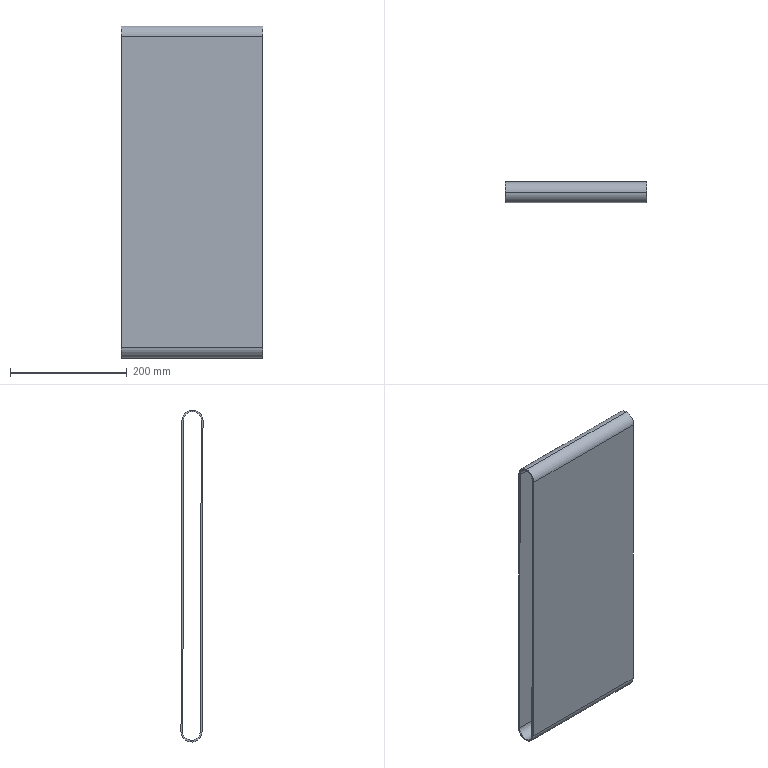Component | SolidWorks | Part7-1 | 1 solid | 12 faces | box 242 x 37.75 x 568.56 mm | volume 848551 mm3 | cylinder 6 | plane 6 | commonest cylinder face diameters 30 x3 36 x3
build123d program:
from build123d import *

# Parameters (mm, degrees)
EXTRUDE_THIN1_DEPTH = 121


with BuildPart() as part:
    # Sketch1 → Extrude-Thin1 (new, symmetric)
    with BuildSketch(Plane.XY):
        with BuildLine():
            Line((2289.339, 197.876), (1756.777, 196.124))
            ThreePointArc((1756.777, 196.124), (1738.718, 214.065), (1756.658, 232.124))
            Line((1756.658, 232.124), (2289.22, 233.876))
            ThreePointArc((2289.22, 233.876), (2307.279, 215.935), (2289.339, 197.876))
        make_face()
        with BuildLine():
            Line((2289.329, 200.876), (1756.767, 199.124))
            ThreePointArc((1756.767, 199.124), (1741.718, 214.075), (1756.668, 229.124))
            Line((1756.668, 229.124), (2289.23, 230.876))
            ThreePointArc((2289.23, 230.876), (2304.279, 215.925), (2289.329, 200.876))
        make_face(mode=Mode.SUBTRACT)
    extrude(amount=EXTRUDE_THIN1_DEPTH, both=True)


solid = part.part

# Placed as in the assembly
solid = solid.moved(Location((0, 0, -143.093), (0, 90, 0)))
STEP:
#1=CARTESIAN_POINT('',(4.764,9.021,-74.794));
#2=VERTEX_POINT('',#1);
#3=CARTESIAN_POINT('',(4.764,8.43,-74.205));
#4=VERTEX_POINT('',#3);
#5=CARTESIAN_POINT('',(4.764,8.43,-74.796));
#6=DIRECTION('',(1.,0.,0.));
#7=DIRECTION('',(0.,0.,-1.));
#8=AXIS2_PLACEMENT_3D('',#5,#6,#7);
#9=CIRCLE('',#8,0.5906);
#10=EDGE_CURVE('',#2,#4,#9,.T.);
#11=ORIENTED_EDGE('',*,*,#10,.T.);
#12=CARTESIAN_POINT('',(-4.764,8.43,-74.205));
#13=VERTEX_POINT('',#12);
#14=CARTESIAN_POINT('',(4.764,8.43,-74.205));
#15=DIRECTION('',(-1.,0.,0.));
#16=VECTOR('',#15,39.37);
#17=LINE('',#14,#16);
#18=EDGE_CURVE('',#4,#13,#17,.T.);
#19=ORIENTED_EDGE('',*,*,#18,.T.);
#20=CARTESIAN_POINT('',(-4.764,9.021,-74.794));
#21=VERTEX_POINT('',#20);
#22=CARTESIAN_POINT('',(-4.764,8.43,-74.796));
#23=DIRECTION('',(1.,0.,0.));
#24=DIRECTION('',(0.,0.,-1.));
#25=AXIS2_PLACEMENT_3D('',#22,#23,#24);
#26=CIRCLE('',#25,0.5906);
#27=EDGE_CURVE('',#21,#13,#26,.T.);
#28=ORIENTED_EDGE('',*,*,#27,.F.);
#29=CARTESIAN_POINT('',(4.764,9.021,-74.794));
#30=DIRECTION('',(-1.,0.,0.));
#31=VECTOR('',#30,39.37);
#32=LINE('',#29,#31);
#33=EDGE_CURVE('',#2,#21,#32,.T.);
#34=ORIENTED_EDGE('',*,*,#33,.F.);
#35=EDGE_LOOP('',(#11,#19,#28,#34));
#36=FACE_OUTER_BOUND('',#35,.T.);
#37=CARTESIAN_POINT('',(4.764,8.43,-74.796));
#38=DIRECTION('',(-1.,0.,0.));
#39=DIRECTION('',(0.,0.,1.));
#40=AXIS2_PLACEMENT_3D('',#37,#38,#39);
#41=CYLINDRICAL_SURFACE('',#40,0.5906);
#42=ADVANCED_FACE('',(#36),#41,.F.);
#43=CARTESIAN_POINT('',(4.764,8.43,-74.087));
#44=VERTEX_POINT('',#43);
#45=CARTESIAN_POINT('',(4.764,7.721,-74.798));
#46=VERTEX_POINT('',#45);
#47=CARTESIAN_POINT('',(4.764,8.43,-74.796));
#48=DIRECTION('',(1.,0.,0.));
#49=DIRECTION('',(0.,0.,-1.));
#50=AXIS2_PLACEMENT_3D('',#47,#48,#49);
#51=CIRCLE('',#50,0.7087);
#52=EDGE_CURVE('',#44,#46,#51,.T.);
#53=ORIENTED_EDGE('',*,*,#52,.F.);
#54=CARTESIAN_POINT('',(-4.764,8.43,-74.087));
#55=VERTEX_POINT('',#54);
#56=CARTESIAN_POINT('',(4.764,8.43,-74.087));
#57=DIRECTION('',(-1.,0.,0.));
#58=VECTOR('',#57,39.37);
#59=LINE('',#56,#58);
#60=EDGE_CURVE('',#44,#55,#59,.T.);
#61=ORIENTED_EDGE('',*,*,#60,.T.);
#62=CARTESIAN_POINT('',(-4.764,7.721,-74.798));
#63=VERTEX_POINT('',#62);
#64=CARTESIAN_POINT('',(-4.764,8.43,-74.796));
#65=DIRECTION('',(1.,0.,0.));
#66=DIRECTION('',(0.,0.,-1.));
#67=AXIS2_PLACEMENT_3D('',#64,#65,#66);
#68=CIRCLE('',#67,0.7087);
#69=EDGE_CURVE('',#55,#63,#68,.T.);
#70=ORIENTED_EDGE('',*,*,#69,.T.);
#71=CARTESIAN_POINT('',(4.764,7.721,-74.798));
#72=DIRECTION('',(-1.,0.,0.));
#73=VECTOR('',#72,39.37);
#74=LINE('',#71,#73);
#75=EDGE_CURVE('',#46,#63,#74,.T.);
#76=ORIENTED_EDGE('',*,*,#75,.F.);
#77=EDGE_LOOP('',(#53,#61,#70,#76));
#78=FACE_OUTER_BOUND('',#77,.T.);
#79=CARTESIAN_POINT('',(4.764,8.43,-74.796));
#80=DIRECTION('',(-1.,0.,0.));
#81=DIRECTION('',(0.,0.,1.));
#82=AXIS2_PLACEMENT_3D('',#79,#80,#81);
#83=CYLINDRICAL_SURFACE('',#82,0.7087);
#84=ADVANCED_FACE('',(#78),#83,.T.);
#85=CARTESIAN_POINT('',(-4.764,7.79,-95.765));
#86=VERTEX_POINT('',#85);
#87=CARTESIAN_POINT('',(-4.764,7.494,-5.609));
#88=DIRECTION('',(0.,-0.003289,1.));
#89=VECTOR('',#88,39.37);
#90=LINE('',#87,#89);
#91=EDGE_CURVE('',#86,#63,#90,.T.);
#92=ORIENTED_EDGE('',*,*,#91,.F.);
#93=CARTESIAN_POINT('',(4.764,7.79,-95.765));
#94=VERTEX_POINT('',#93);
#95=CARTESIAN_POINT('',(4.764,7.79,-95.765));
#96=DIRECTION('',(-1.,0.,0.));
#97=VECTOR('',#96,39.37);
#98=LINE('',#95,#97);
#99=EDGE_CURVE('',#94,#86,#98,.T.);
#100=ORIENTED_EDGE('',*,*,#99,.F.);
#101=CARTESIAN_POINT('',(4.764,7.494,-5.609));
#102=DIRECTION('',(0.,-0.003289,1.));
#103=VECTOR('',#102,39.37);
#104=LINE('',#101,#103);
#105=EDGE_CURVE('',#94,#46,#104,.T.);
#106=ORIENTED_EDGE('',*,*,#105,.T.);
#107=ORIENTED_EDGE('',*,*,#75,.T.);
#108=EDGE_LOOP('',(#92,#100,#106,#107));
#109=FACE_OUTER_BOUND('',#108,.T.);
#110=CARTESIAN_POINT('',(4.764,7.494,-5.609));
#111=DIRECTION('',(0.,-1.,-0.003289));
#112=DIRECTION('',(0.,0.003289,-1.));
#113=AXIS2_PLACEMENT_3D('',#110,#111,#112);
#114=PLANE('',#113);
#115=ADVANCED_FACE('',(#109),#114,.T.);
#116=CARTESIAN_POINT('',(-4.764,9.208,-95.76));
#117=VERTEX_POINT('',#116);
#118=CARTESIAN_POINT('',(-4.764,8.499,-95.763));
#119=DIRECTION('',(1.,0.,0.));
#120=DIRECTION('',(0.,0.,-1.));
#121=AXIS2_PLACEMENT_3D('',#118,#119,#120);
#122=CIRCLE('',#121,0.7087);
#123=EDGE_CURVE('',#86,#117,#122,.T.);
#124=ORIENTED_EDGE('',*,*,#123,.T.);
#125=CARTESIAN_POINT('',(4.764,9.208,-95.76));
#126=VERTEX_POINT('',#125);
#127=CARTESIAN_POINT('',(4.764,9.208,-95.76));
#128=DIRECTION('',(-1.,0.,0.));
#129=VECTOR('',#128,39.37);
#130=LINE('',#127,#129);
#131=EDGE_CURVE('',#126,#117,#130,.T.);
#132=ORIENTED_EDGE('',*,*,#131,.F.);
#133=CARTESIAN_POINT('',(4.764,8.499,-95.763));
#134=DIRECTION('',(1.,0.,0.));
#135=DIRECTION('',(0.,0.,-1.));
#136=AXIS2_PLACEMENT_3D('',#133,#134,#135);
#137=CIRCLE('',#136,0.7087);
#138=EDGE_CURVE('',#94,#126,#137,.T.);
#139=ORIENTED_EDGE('',*,*,#138,.F.);
#140=ORIENTED_EDGE('',*,*,#99,.T.);
#141=EDGE_LOOP('',(#124,#132,#139,#140));
#142=FACE_OUTER_BOUND('',#141,.T.);
#143=CARTESIAN_POINT('',(4.764,8.499,-95.763));
#144=DIRECTION('',(-1.,0.,0.));
#145=DIRECTION('',(0.,0.,1.));
#146=AXIS2_PLACEMENT_3D('',#143,#144,#145);
#147=CYLINDRICAL_SURFACE('',#146,0.7087);
#148=ADVANCED_FACE('',(#142),#147,.T.);
#149=CARTESIAN_POINT('',(-4.764,9.139,-74.793));
#150=VERTEX_POINT('',#149);
#151=CARTESIAN_POINT('',(-4.764,8.911,-5.604));
#152=DIRECTION('',(0.,0.003289,-1.));
#153=VECTOR('',#152,39.37);
#154=LINE('',#151,#153);
#155=EDGE_CURVE('',#150,#117,#154,.T.);
#156=ORIENTED_EDGE('',*,*,#155,.F.);
#157=CARTESIAN_POINT('',(4.764,9.139,-74.793));
#158=VERTEX_POINT('',#157);
#159=CARTESIAN_POINT('',(4.764,9.139,-74.793));
#160=DIRECTION('',(-1.,0.,0.));
#161=VECTOR('',#160,39.37);
#162=LINE('',#159,#161);
#163=EDGE_CURVE('',#158,#150,#162,.T.);
#164=ORIENTED_EDGE('',*,*,#163,.F.);
#165=CARTESIAN_POINT('',(4.764,8.911,-5.604));
#166=DIRECTION('',(0.,0.003289,-1.));
#167=VECTOR('',#166,39.37);
#168=LINE('',#165,#167);
#169=EDGE_CURVE('',#158,#126,#168,.T.);
#170=ORIENTED_EDGE('',*,*,#169,.T.);
#171=ORIENTED_EDGE('',*,*,#131,.T.);
#172=EDGE_LOOP('',(#156,#164,#170,#171));
#173=FACE_OUTER_BOUND('',#172,.T.);
#174=CARTESIAN_POINT('',(4.764,8.911,-5.604));
#175=DIRECTION('',(0.,1.,0.003289));
#176=DIRECTION('',(0.,-0.003289,1.));
#177=AXIS2_PLACEMENT_3D('',#174,#175,#176);
#178=PLANE('',#177);
#179=ADVANCED_FACE('',(#173),#178,.T.);
#180=ORIENTED_EDGE('',*,*,#60,.F.);
#181=CARTESIAN_POINT('',(4.764,8.43,-74.796));
#182=DIRECTION('',(1.,0.,0.));
#183=DIRECTION('',(0.,0.,-1.));
#184=AXIS2_PLACEMENT_3D('',#181,#182,#183);
#185=CIRCLE('',#184,0.7087);
#186=EDGE_CURVE('',#158,#44,#185,.T.);
#187=ORIENTED_EDGE('',*,*,#186,.F.);
#188=ORIENTED_EDGE('',*,*,#163,.T.);
#189=CARTESIAN_POINT('',(-4.764,8.43,-74.796));
#190=DIRECTION('',(1.,0.,0.));
#191=DIRECTION('',(0.,0.,-1.));
#192=AXIS2_PLACEMENT_3D('',#189,#190,#191);
#193=CIRCLE('',#192,0.7087);
#194=EDGE_CURVE('',#150,#55,#193,.T.);
#195=ORIENTED_EDGE('',*,*,#194,.T.);
#196=EDGE_LOOP('',(#180,#187,#188,#195));
#197=FACE_OUTER_BOUND('',#196,.T.);
#198=CARTESIAN_POINT('',(4.764,8.43,-74.796));
#199=DIRECTION('',(-1.,0.,0.));
#200=DIRECTION('',(0.,0.,1.));
#201=AXIS2_PLACEMENT_3D('',#198,#199,#200);
#202=CYLINDRICAL_SURFACE('',#201,0.7087);
#203=ADVANCED_FACE('',(#197),#202,.T.);
#204=CARTESIAN_POINT('',(4.764,7.909,-95.765));
#205=VERTEX_POINT('',#204);
#206=CARTESIAN_POINT('',(4.764,7.84,-74.798));
#207=VERTEX_POINT('',#206);
#208=CARTESIAN_POINT('',(4.764,7.612,-5.609));
#209=DIRECTION('',(0.,-0.003289,1.));
#210=VECTOR('',#209,39.37);
#211=LINE('',#208,#210);
#212=EDGE_CURVE('',#205,#207,#211,.T.);
#213=ORIENTED_EDGE('',*,*,#212,.T.);
#214=CARTESIAN_POINT('',(4.764,8.43,-74.796));
#215=DIRECTION('',(1.,0.,0.));
#216=DIRECTION('',(0.,0.,-1.));
#217=AXIS2_PLACEMENT_3D('',#214,#215,#216);
#218=CIRCLE('',#217,0.5906);
#219=EDGE_CURVE('',#4,#207,#218,.T.);
#220=ORIENTED_EDGE('',*,*,#219,.F.);
#221=ORIENTED_EDGE('',*,*,#10,.F.);
#222=CARTESIAN_POINT('',(4.764,9.09,-95.761));
#223=VERTEX_POINT('',#222);
#224=CARTESIAN_POINT('',(4.764,8.793,-5.605));
#225=DIRECTION('',(0.,0.003289,-1.));
#226=VECTOR('',#225,39.37);
#227=LINE('',#224,#226);
#228=EDGE_CURVE('',#2,#223,#227,.T.);
#229=ORIENTED_EDGE('',*,*,#228,.T.);
#230=CARTESIAN_POINT('',(4.764,8.499,-95.763));
#231=DIRECTION('',(1.,0.,0.));
#232=DIRECTION('',(0.,0.,-1.));
#233=AXIS2_PLACEMENT_3D('',#230,#231,#232);
#234=CIRCLE('',#233,0.5906);
#235=EDGE_CURVE('',#205,#223,#234,.T.);
#236=ORIENTED_EDGE('',*,*,#235,.F.);
#237=EDGE_LOOP('',(#213,#220,#221,#229,#236));
#238=FACE_BOUND('',#237,.T.);
#239=ORIENTED_EDGE('',*,*,#105,.F.);
#240=ORIENTED_EDGE('',*,*,#138,.T.);
#241=ORIENTED_EDGE('',*,*,#169,.F.);
#242=ORIENTED_EDGE('',*,*,#186,.T.);
#243=ORIENTED_EDGE('',*,*,#52,.T.);
#244=EDGE_LOOP('',(#239,#240,#241,#242,#243));
#245=FACE_OUTER_BOUND('',#244,.T.);
#246=CARTESIAN_POINT('',(4.764,8.43,-74.796));
#247=DIRECTION('',(1.,0.,0.));
#248=DIRECTION('',(0.,0.,-1.));
#249=AXIS2_PLACEMENT_3D('',#246,#247,#248);
#250=PLANE('',#249);
#251=ADVANCED_FACE('',(#238,#245),#250,.T.);
#252=ORIENTED_EDGE('',*,*,#27,.T.);
#253=CARTESIAN_POINT('',(-4.764,7.84,-74.798));
#254=VERTEX_POINT('',#253);
#255=CARTESIAN_POINT('',(-4.764,8.43,-74.796));
#256=DIRECTION('',(1.,0.,0.));
#257=DIRECTION('',(0.,0.,-1.));
#258=AXIS2_PLACEMENT_3D('',#255,#256,#257);
#259=CIRCLE('',#258,0.5906);
#260=EDGE_CURVE('',#13,#254,#259,.T.);
#261=ORIENTED_EDGE('',*,*,#260,.T.);
#262=CARTESIAN_POINT('',(-4.764,7.909,-95.765));
#263=VERTEX_POINT('',#262);
#264=CARTESIAN_POINT('',(-4.764,7.612,-5.609));
#265=DIRECTION('',(0.,-0.003289,1.));
#266=VECTOR('',#265,39.37);
#267=LINE('',#264,#266);
#268=EDGE_CURVE('',#263,#254,#267,.T.);
#269=ORIENTED_EDGE('',*,*,#268,.F.);
#270=CARTESIAN_POINT('',(-4.764,9.09,-95.761));
#271=VERTEX_POINT('',#270);
#272=CARTESIAN_POINT('',(-4.764,8.499,-95.763));
#273=DIRECTION('',(1.,0.,0.));
#274=DIRECTION('',(0.,0.,-1.));
#275=AXIS2_PLACEMENT_3D('',#272,#273,#274);
#276=CIRCLE('',#275,0.5906);
#277=EDGE_CURVE('',#263,#271,#276,.T.);
#278=ORIENTED_EDGE('',*,*,#277,.T.);
#279=CARTESIAN_POINT('',(-4.764,8.793,-5.605));
#280=DIRECTION('',(0.,0.003289,-1.));
#281=VECTOR('',#280,39.37);
#282=LINE('',#279,#281);
#283=EDGE_CURVE('',#21,#271,#282,.T.);
#284=ORIENTED_EDGE('',*,*,#283,.F.);
#285=EDGE_LOOP('',(#252,#261,#269,#278,#284));
#286=FACE_BOUND('',#285,.T.);
#287=ORIENTED_EDGE('',*,*,#91,.T.);
#288=ORIENTED_EDGE('',*,*,#69,.F.);
#289=ORIENTED_EDGE('',*,*,#194,.F.);
#290=ORIENTED_EDGE('',*,*,#155,.T.);
#291=ORIENTED_EDGE('',*,*,#123,.F.);
#292=EDGE_LOOP('',(#287,#288,#289,#290,#291));
#293=FACE_OUTER_BOUND('',#292,.T.);
#294=CARTESIAN_POINT('',(-4.764,8.43,-74.796));
#295=DIRECTION('',(1.,0.,0.));
#296=DIRECTION('',(0.,0.,-1.));
#297=AXIS2_PLACEMENT_3D('',#294,#295,#296);
#298=PLANE('',#297);
#299=ADVANCED_FACE('',(#286,#293),#298,.F.);
#300=ORIENTED_EDGE('',*,*,#268,.T.);
#301=CARTESIAN_POINT('',(4.764,7.84,-74.798));
#302=DIRECTION('',(-1.,0.,0.));
#303=VECTOR('',#302,39.37);
#304=LINE('',#301,#303);
#305=EDGE_CURVE('',#207,#254,#304,.T.);
#306=ORIENTED_EDGE('',*,*,#305,.F.);
#307=ORIENTED_EDGE('',*,*,#212,.F.);
#308=CARTESIAN_POINT('',(4.764,7.909,-95.765));
#309=DIRECTION('',(-1.,0.,0.));
#310=VECTOR('',#309,39.37);
#311=LINE('',#308,#310);
#312=EDGE_CURVE('',#205,#263,#311,.T.);
#313=ORIENTED_EDGE('',*,*,#312,.T.);
#314=EDGE_LOOP('',(#300,#306,#307,#313));
#315=FACE_OUTER_BOUND('',#314,.T.);
#316=CARTESIAN_POINT('',(4.764,7.612,-5.609));
#317=DIRECTION('',(0.,-1.,-0.003289));
#318=DIRECTION('',(0.,0.003289,-1.));
#319=AXIS2_PLACEMENT_3D('',#316,#317,#318);
#320=PLANE('',#319);
#321=ADVANCED_FACE('',(#315),#320,.F.);
#322=ORIENTED_EDGE('',*,*,#277,.F.);
#323=ORIENTED_EDGE('',*,*,#312,.F.);
#324=ORIENTED_EDGE('',*,*,#235,.T.);
#325=CARTESIAN_POINT('',(4.764,9.09,-95.761));
#326=DIRECTION('',(-1.,0.,0.));
#327=VECTOR('',#326,39.37);
#328=LINE('',#325,#327);
#329=EDGE_CURVE('',#223,#271,#328,.T.);
#330=ORIENTED_EDGE('',*,*,#329,.T.);
#331=EDGE_LOOP('',(#322,#323,#324,#330));
#332=FACE_OUTER_BOUND('',#331,.T.);
#333=CARTESIAN_POINT('',(4.764,8.499,-95.763));
#334=DIRECTION('',(-1.,0.,0.));
#335=DIRECTION('',(0.,0.,1.));
#336=AXIS2_PLACEMENT_3D('',#333,#334,#335);
#337=CYLINDRICAL_SURFACE('',#336,0.5906);
#338=ADVANCED_FACE('',(#332),#337,.F.);
#339=ORIENTED_EDGE('',*,*,#283,.T.);
#340=ORIENTED_EDGE('',*,*,#329,.F.);
#341=ORIENTED_EDGE('',*,*,#228,.F.);
#342=ORIENTED_EDGE('',*,*,#33,.T.);
#343=EDGE_LOOP('',(#339,#340,#341,#342));
#344=FACE_OUTER_BOUND('',#343,.T.);
#345=CARTESIAN_POINT('',(4.764,8.793,-5.605));
#346=DIRECTION('',(0.,1.,0.003289));
#347=DIRECTION('',(0.,-0.003289,1.));
#348=AXIS2_PLACEMENT_3D('',#345,#346,#347);
#349=PLANE('',#348);
#350=ADVANCED_FACE('',(#344),#349,.F.);
#351=ORIENTED_EDGE('',*,*,#18,.F.);
#352=ORIENTED_EDGE('',*,*,#219,.T.);
#353=ORIENTED_EDGE('',*,*,#305,.T.);
#354=ORIENTED_EDGE('',*,*,#260,.F.);
#355=EDGE_LOOP('',(#351,#352,#353,#354));
#356=FACE_OUTER_BOUND('',#355,.T.);
#357=CARTESIAN_POINT('',(4.764,8.43,-74.796));
#358=DIRECTION('',(-1.,0.,0.));
#359=DIRECTION('',(0.,0.,1.));
#360=AXIS2_PLACEMENT_3D('',#357,#358,#359);
#361=CYLINDRICAL_SURFACE('',#360,0.5906);
#362=ADVANCED_FACE('',(#356),#361,.F.);
#363=CLOSED_SHELL('',(#42,#84,#115,#148,#179,#203,#251,#299,#321,#338,#350,#362));
#364=MANIFOLD_SOLID_BREP('',#363);
#365=CARTESIAN_POINT('',(0.,0.,0.));
#366=DIRECTION('',(0.,0.,1.));
#367=DIRECTION('',(1.,0.,0.));
#368=AXIS2_PLACEMENT_3D('',#365,#366,#367);
#369=(LENGTH_UNIT()NAMED_UNIT(*)SI_UNIT($,.METRE.));
#370=LENGTH_MEASURE_WITH_UNIT(LENGTH_MEASURE(0.0254),#369);
#371=DIMENSIONAL_EXPONENTS(1.,0.,0.,0.,0.,0.,0.);
#372=(CONVERSION_BASED_UNIT('',#370)LENGTH_UNIT()NAMED_UNIT(#371));
#373=UNCERTAINTY_MEASURE_WITH_UNIT(LENGTH_MEASURE(0.00001),#372,'','');
#374=(NAMED_UNIT(*)PLANE_ANGLE_UNIT()SI_UNIT($,.RADIAN.));
#375=(NAMED_UNIT(*)SI_UNIT($,.STERADIAN.)SOLID_ANGLE_UNIT());
#376=(GEOMETRIC_REPRESENTATION_CONTEXT(3)GLOBAL_UNCERTAINTY_ASSIGNED_CONTEXT((#373))GLOBAL_UNIT_ASSIGNED_CONTEXT((#372,#374,#375))REPRESENTATION_CONTEXT('',''));
#377=ADVANCED_BREP_SHAPE_REPRESENTATION('',(#364,#368),#376);
#378=COLOUR_RGB('',0.7922,0.8196,0.9333);
#379=FILL_AREA_STYLE_COLOUR('',#378);
#380=FILL_AREA_STYLE('',(#379));
#381=SURFACE_STYLE_FILL_AREA(#380);
#382=SURFACE_SIDE_STYLE('',(#381));
#383=SURFACE_STYLE_USAGE(.BOTH.,#382);
#384=PRESENTATION_STYLE_ASSIGNMENT((#383));
#385=STYLED_ITEM('',(#384),#364);
#386=PRESENTATION_LAYER_ASSIGNMENT('','',(#385));
#387=(LENGTH_UNIT()NAMED_UNIT(*)SI_UNIT($,.METRE.));
#388=LENGTH_MEASURE_WITH_UNIT(LENGTH_MEASURE(0.0254),#387);
#389=DIMENSIONAL_EXPONENTS(1.,0.,0.,0.,0.,0.,0.);
#390=(CONVERSION_BASED_UNIT('',#388)LENGTH_UNIT()NAMED_UNIT(#389));
#391=UNCERTAINTY_MEASURE_WITH_UNIT(LENGTH_MEASURE(0.00001),#390,'','');
#392=(NAMED_UNIT(*)PLANE_ANGLE_UNIT()SI_UNIT($,.RADIAN.));
#393=(NAMED_UNIT(*)SI_UNIT($,.STERADIAN.)SOLID_ANGLE_UNIT());
#394=(GEOMETRIC_REPRESENTATION_CONTEXT(3)GLOBAL_UNCERTAINTY_ASSIGNED_CONTEXT((#391))GLOBAL_UNIT_ASSIGNED_CONTEXT((#390,#392,#393))REPRESENTATION_CONTEXT('',''));
#395=MECHANICAL_DESIGN_GEOMETRIC_PRESENTATION_REPRESENTATION('',(#385),#394);